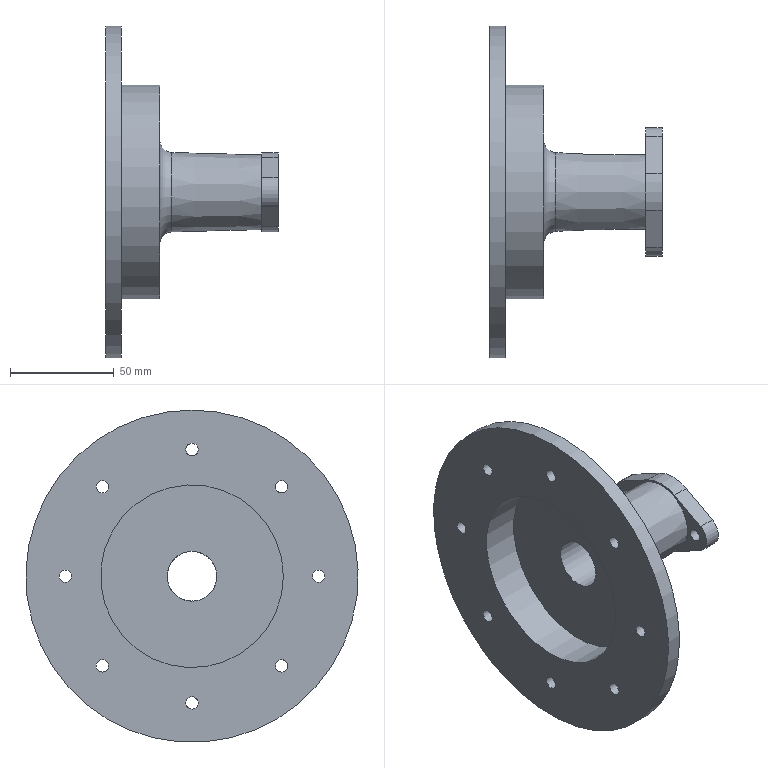Component | NX | REAR_CYLINDER_HEAD | 1 solid | 32 faces | volume 225395 mm3 | cylinder 19 | plane 11 | cone 1 | torus 1 | commonest cylinder face diameters 6 x10 16 x2 38 x2 103 x1 160 x1 27 x1 24 x1 88 x1